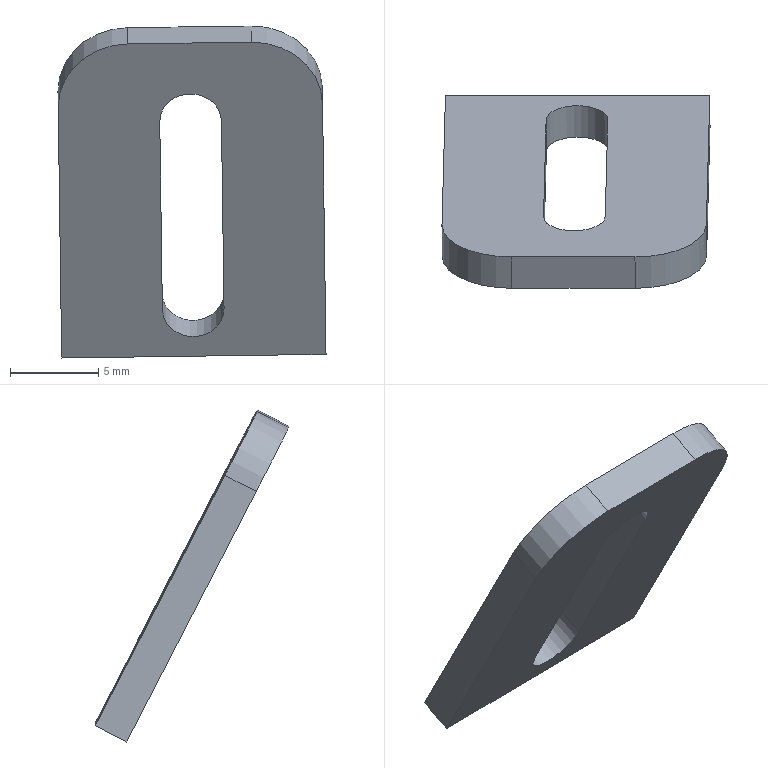Component | SolidWorks | 2018SOLIDWORKS1400000011-1 | 1 solid | 12 faces | volume 483 mm3 | plane 8 | cylinder 4 | commonest cylinder face diameters 3.5 x2 8 x2 | material Black POM